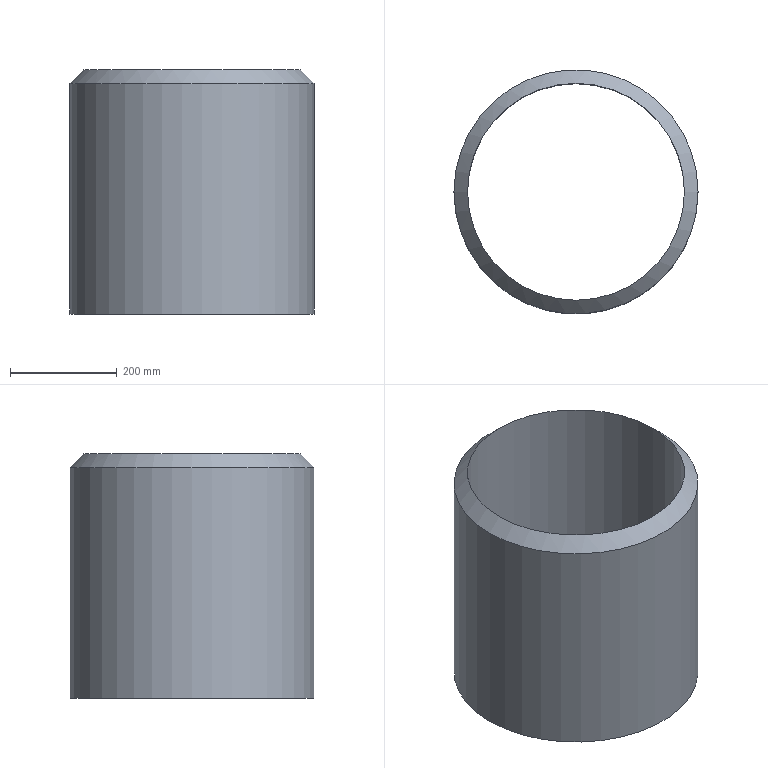Component | NX | 8 | 1 solid | 4 faces | volume 15307160 mm3 | cylinder 2 | plane 1 | cone 1 | commonest cylinder face diameters 457.2 x1 406.4 x1